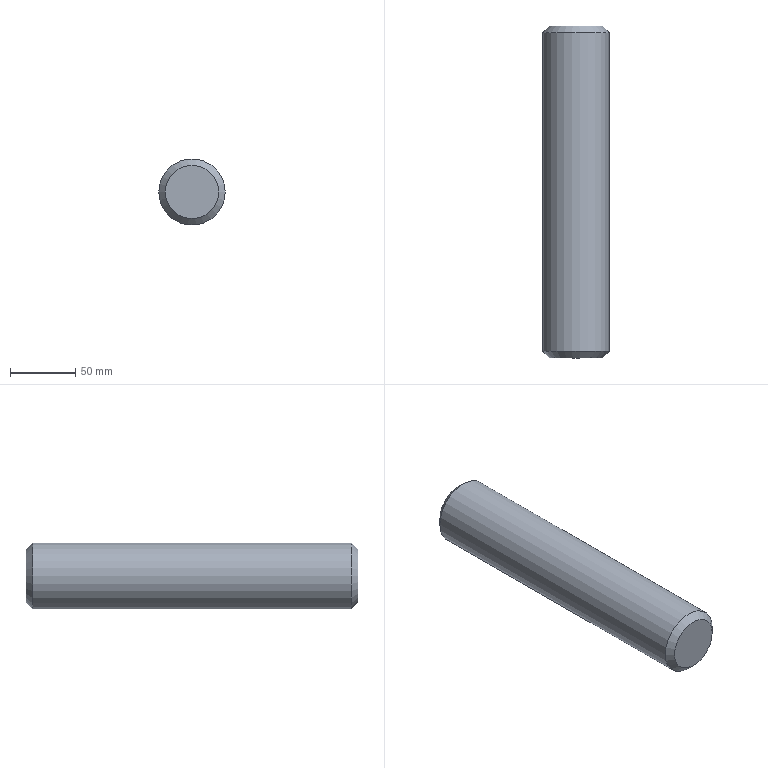Component | NX | PIN_254 | 1 solid | 5 faces | volume 511087 mm3 | plane 2 | cone 2 | cylinder 1 | commonest cylinder face diameters 50.8 x1